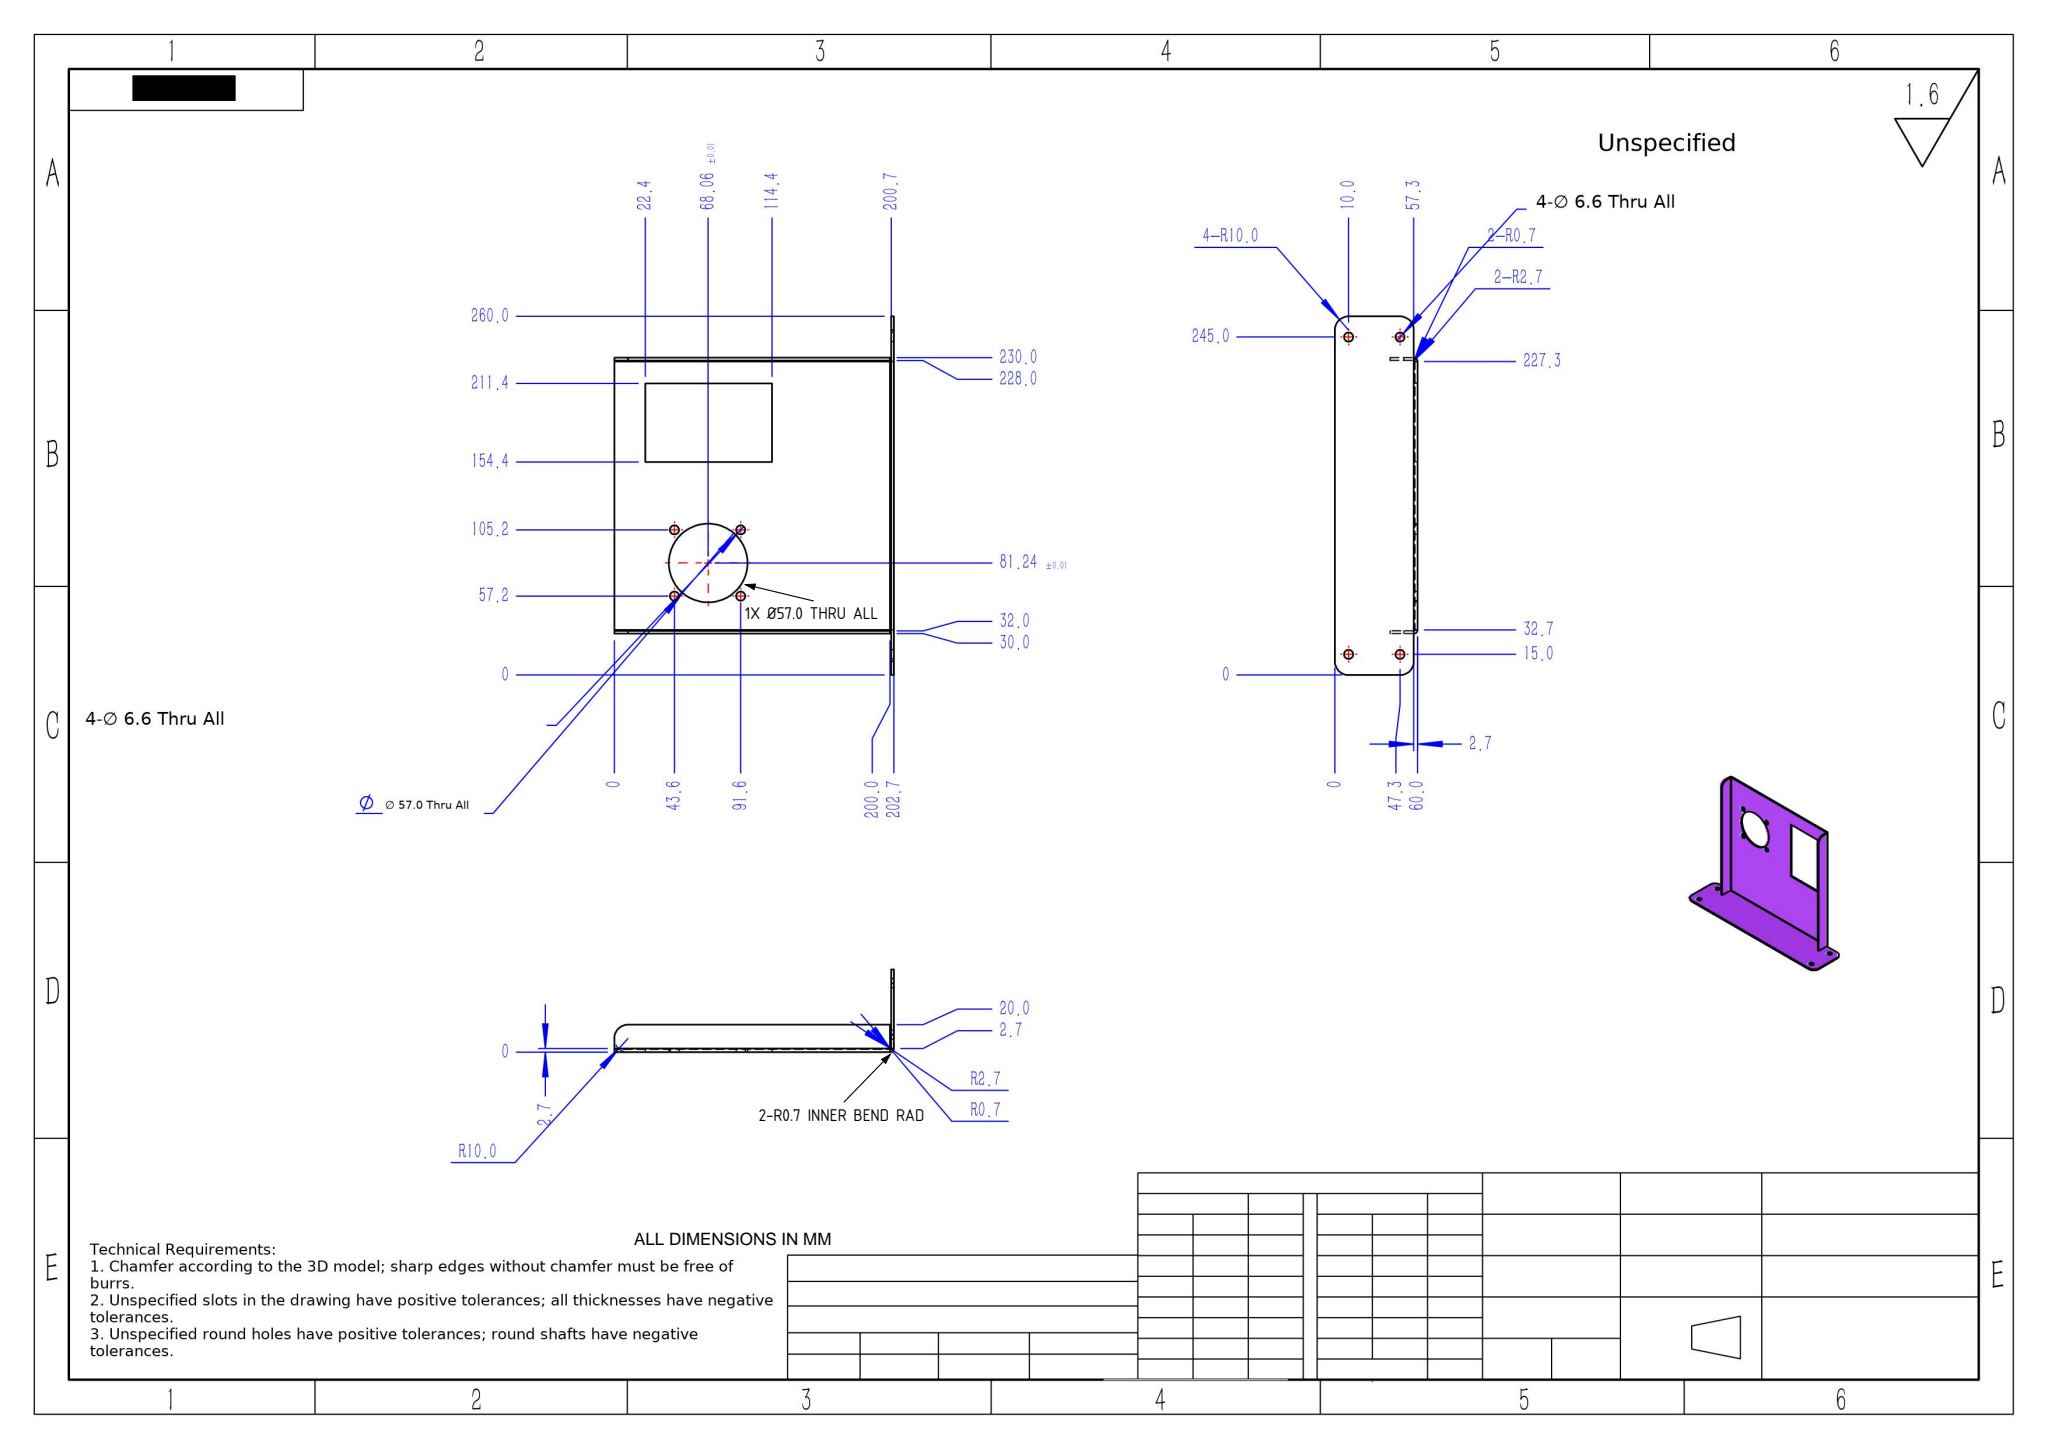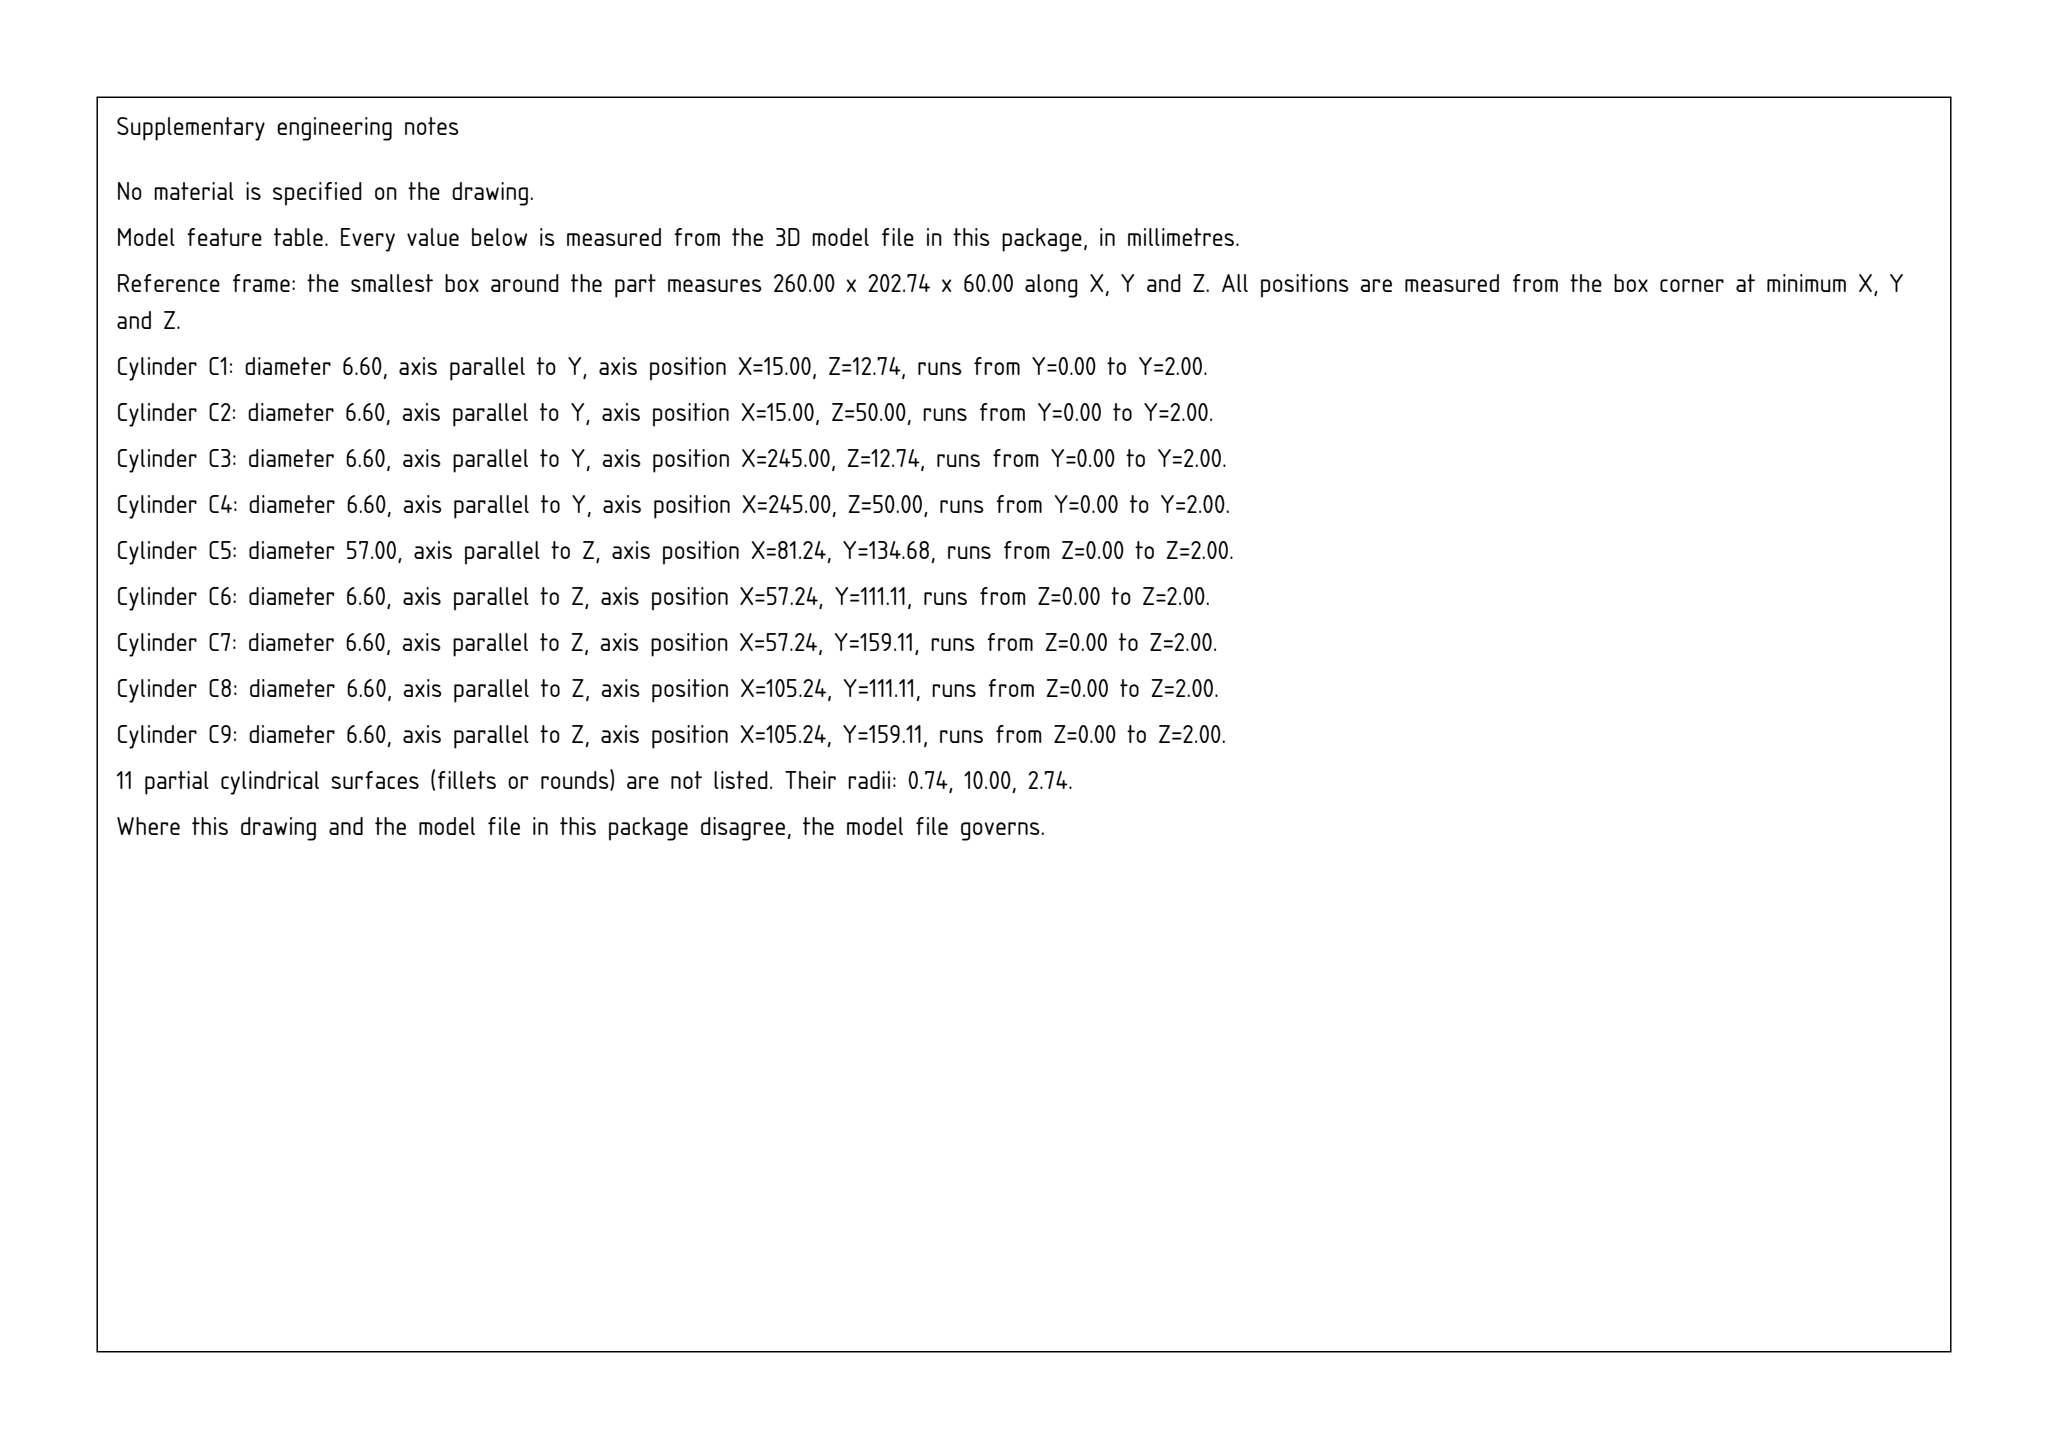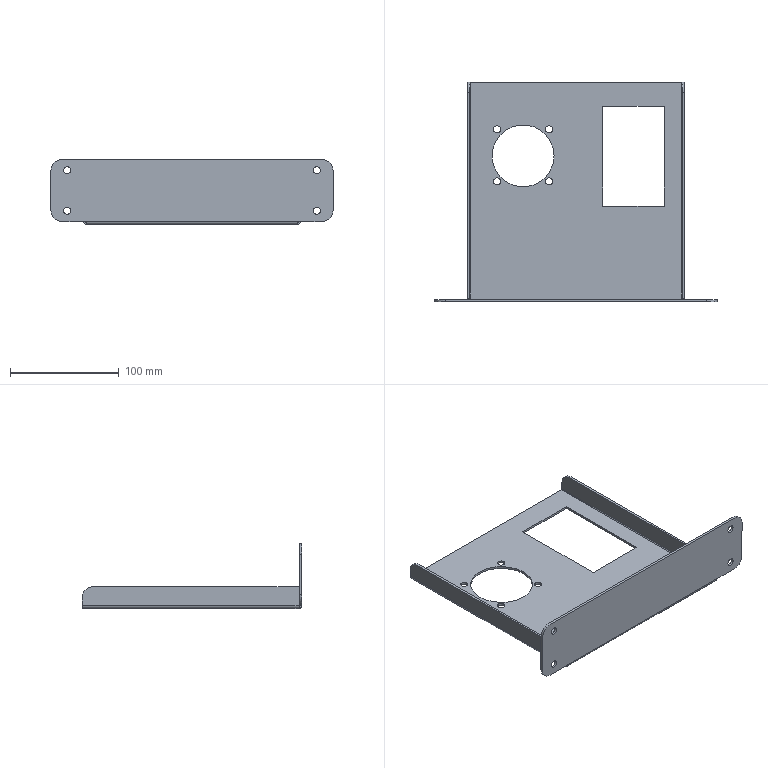Part | SolidWorks | mm | 1 solid | 60 faces | box 260 x 202.74 x 60 mm | volume 108246 mm3 | cylinder 30 | plane 30 | commonest cylinder face diameters 6.6 x16 20 x6 5.473 x3 1.473 x3 57 x2
Drawing notes:
FRONT VIEW: 1X Ø57.0 THRU ALL, CTR 81.24 x 134.7 (NOT 4X Ø6.6) | from the solid: hole/bore dia 57.0 axis z at [81.2,134.7], from 0.0 to 2.0 (2 THK plate); separate 4X dia 6.6 bores at x57.2/105.2, y111.1/159.1
2-R0.7 INNER BEND RAD AT 32.7 & 227.3 | from the solid: 2X concave arc dia 1.47 (R0.735) axis y at [227.3,-,2.7] and [32.7,-,2.7], 90 deg, y 2.7 to 202.7; paired with 2X convex dia 5.47 (R2.7)